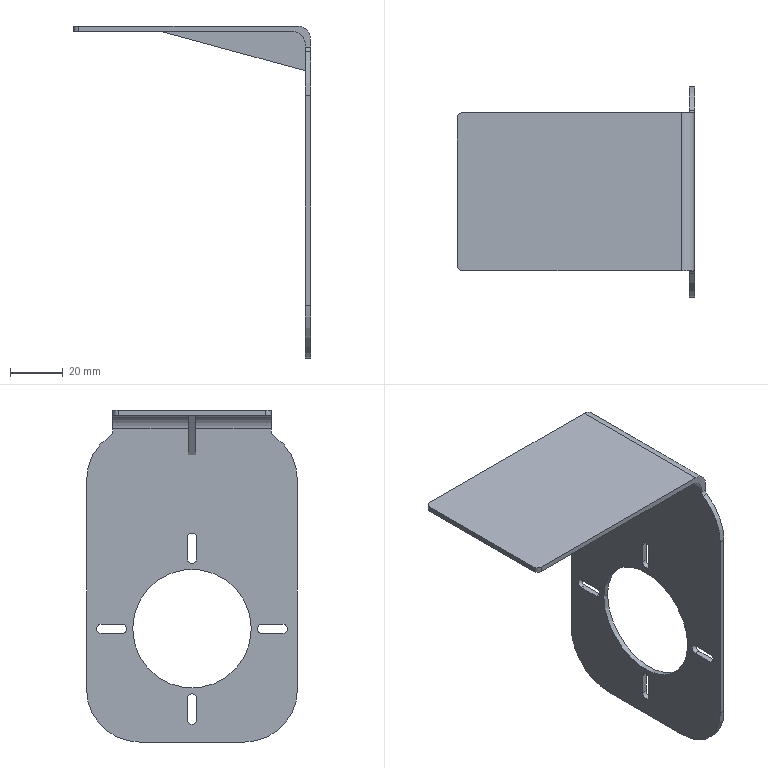Component | SolidWorks | ImagingSystem-1111-1_123456789-DL-OP20-ST12--004-1111-1 | 1 solid | 43 faces | box 90 x 80 x 126 mm | volume 27547 mm3 | cylinder 22 | plane 21 | commonest cylinder face diameters 3.5 x9 4 x4 40 x4 10 x3 45 x2 | material AL6061
build123d program:
from build123d import *

# Parameters (mm, degrees)
SKETCH1_W                  = 80
SKETCH1_H                  = 126
BOSS_EXTRUDE1_DEPTH        = 30
SKETCH2_W                  = 20
SKETCH2_H                  = 116
CUT_EXTRUDE1_DEPTH         = 152.331
F_25_0_25_DIAMETER_HOLE1_D = 45
CHAMFER1_SIZE              = 2
SKETCH9_W                  = 30
SKETCH9_H                  = 10
CUT_EXTRUDE3_DEPTH         = 10
SKETCH10_W                 = 30
SKETCH10_H                 = 10
CUT_EXTRUDE4_DEPTH         = 10
MOVE_FACE1_BY              = 3
MOVE_FACE1_2_BY            = 3
SKETCH15_W                 = 3
SKETCH15_H                 = 30
BOSS_EXTRUDE2_DEPTH        = 3
F_3_5_3_5_DIAMETER_HOLE2_D = 3.5
CIRPATTERN1_COUNT          = 4
MOVE_FACE2_BY              = 8
SKETCH22_W                 = 30
SKETCH22_H                 = 3
CUT_EXTRUDE11_DEPTH        = 10
SKETCH23_W                 = 30
SKETCH23_H                 = 3
CUT_EXTRUDE12_DEPTH        = 10
MOVE_FACE4_BY              = 8
FILLET3_R                  = 5
MOVE_FACE6_BY              = 3
MOVE_FACE7_BY              = 3
MOVE_FACE8_BY              = 60
FILLET4_R                  = 2
FILLET8_R                  = 20
BOSS_EXTRUDE7_DEPTH        = 1.5
CUT_EXTRUDE15_DEPTH        = 174.263
CIRPATTERN2_COUNT          = 4


with BuildPart() as part:
    # Sketch1 → Boss-Extrude1 (new body)
    with BuildSketch(Plane.XY.offset(25)):
        with Locations((40, 63)):
            Rectangle(SKETCH1_W, SKETCH1_H)
    extrude(amount=-BOSS_EXTRUDE1_DEPTH)

    # Sketch2 → Cut-Extrude1 (cut, through all)
    with BuildSketch(Plane.ZY):
        with Locations((15, 58)):
            Rectangle(SKETCH2_W, SKETCH2_H)
    extrude(amount=-CUT_EXTRUDE1_DEPTH, mode=Mode.SUBTRACT)

    # 25.0 _25_ Diameter Hole1 (through all)
    with Locations(Plane.XY.offset(5)):
        with Locations((40, 43)):
            Hole(F_25_0_25_DIAMETER_HOLE1_D / 2)

    # Chamfer1
    chamfer1_edges = [part.edges().sort_by_distance(p)[0] for p in [
        (80, 121, 25),
        (0, 121, 25),
    ]]
    chamfer(chamfer1_edges, length=CHAMFER1_SIZE)

    # Sketch9 → Cut-Extrude3 (cut)
    with BuildSketch(Plane(origin=(80, 0, 0), x_dir=(0, 0, -1), z_dir=(1, 0, 0))):
        with Locations((-10, 121)):
            Rectangle(SKETCH9_W, SKETCH9_H)
    extrude(amount=-CUT_EXTRUDE3_DEPTH, mode=Mode.SUBTRACT)

    # Sketch10 → Cut-Extrude4 (cut)
    with BuildSketch(Plane.ZY):
        with Locations((10, 121)):
            Rectangle(SKETCH10_W, SKETCH10_H)
    extrude(amount=-CUT_EXTRUDE4_DEPTH, mode=Mode.SUBTRACT)

    # Move Face1: a face moved outward by 3.0
    extrude(part.faces().sort_by_distance((10, 121, 10))[0], amount=MOVE_FACE1_BY, dir=(-1, 0, 0))

    # Move Face1 2: a face moved outward by 3.0
    extrude(part.faces().sort_by_distance((70, 121, 10))[0], amount=MOVE_FACE1_2_BY, dir=(1, 0, 0))

    # Sketch15 → Boss-Extrude2 (add)
    with BuildSketch(Plane(origin=(0, 126, 0), x_dir=(1, 0, 0), z_dir=(0, 1, 0))):
        with Locations((8.5, -10)):
            Rectangle(SKETCH15_W, SKETCH15_H)
        with Locations((71.5, -10)):
            Rectangle(SKETCH15_W, SKETCH15_H)
    extrude(amount=BOSS_EXTRUDE2_DEPTH)

    # Sketch18 → 3.5 _3.5_ Diameter Hole1 (revolve, cut)
    with BuildSketch(Plane(origin=(40, 77.5, 5), x_dir=(0, -1, 0), z_dir=(1, 0, 0))):
        Polygon((0, 0), (0, 31.052), (1.75, 30), (1.75, 0), align=None)
    f_3_5_3_5_diameter_hole1 = revolve(axis=Axis((40, 77.5, 11.35), (0, 0, -1)), mode=Mode.SUBTRACT)

    # 3.5 _3.5_ Diameter Hole2 (through all)
    with Locations(Plane.XY.offset(5)):
        with Locations((40, 73)):
            f_3_5_3_5_diameter_hole2 = Hole(F_3_5_3_5_DIAMETER_HOLE2_D / 2)

    # CirPattern1: 3.5 _3.5_ Diameter Hole1, 3.5 _3.5_ Diameter Hole2 ×4 about axis
    cirpattern1_axis = Axis((40, 43, 0), (0, 0, 1))
    add([f_3_5_3_5_diameter_hole1.rotate(cirpattern1_axis, i * 360 / CIRPATTERN1_COUNT) for i in range(1, CIRPATTERN1_COUNT)], mode=Mode.SUBTRACT)
    add([f_3_5_3_5_diameter_hole2.rotate(cirpattern1_axis, i * 360 / CIRPATTERN1_COUNT) for i in range(1, CIRPATTERN1_COUNT)], mode=Mode.SUBTRACT)

    # Move Face2: a face moved inward by 8.0
    extrude(part.faces().sort_by_distance((40, 116, 15))[0], amount=MOVE_FACE2_BY, dir=(0, 1, 0), mode=Mode.SUBTRACT)

    # Sketch22 → Cut-Extrude11 (cut)
    with BuildSketch(Plane(origin=(10, 0, 0), x_dir=(0, 0, -1), z_dir=(1, 0, 0))):
        with Locations((-10, 127.5)):
            Rectangle(SKETCH22_W, SKETCH22_H)
    extrude(amount=-CUT_EXTRUDE11_DEPTH, mode=Mode.SUBTRACT)

    # Sketch23 → Cut-Extrude12 (cut)
    with BuildSketch(Plane.ZY.offset(-70)):
        with Locations((10, 127.5)):
            Rectangle(SKETCH23_W, SKETCH23_H)
    extrude(amount=-CUT_EXTRUDE12_DEPTH, mode=Mode.SUBTRACT)

    # Move Face4: a face moved inward by 8.0
    extrude(part.faces().sort_by_distance((60, 62, 5))[0], amount=MOVE_FACE4_BY, dir=(0, 0, -1), mode=Mode.SUBTRACT)

    # Fillet3
    fillet3_edges = [part.edges().sort_by_distance(p)[0] for p in [
        (40, 126, -5),
        (40, 124, -3),
    ]]
    fillet(fillet3_edges, radius=FILLET3_R)

    # Move Face6: a face moved inward by 3.0
    extrude(part.faces().sort_by_distance((7, 125, 10))[0], amount=MOVE_FACE6_BY, dir=(1, 0, 0), mode=Mode.SUBTRACT)

    # Move Face7: a face moved inward by 3.0
    extrude(part.faces().sort_by_distance((73, 125, 10))[0], amount=MOVE_FACE7_BY, dir=(-1, 0, 0), mode=Mode.SUBTRACT)

    # Move Face8: a face moved outward by 60.0
    extrude(part.faces().sort_by_distance((40, 125, 25))[0], amount=MOVE_FACE8_BY, dir=(0, 0, 1))

    # Fillet4
    fillet4_edges = [part.edges().sort_by_distance(p)[0] for p in [
        (70, 125, 85),
        (70, 116, -4),
        (10, 116, -4),
        (10, 125, 85),
    ]]
    fillet(fillet4_edges, radius=FILLET4_R)

    # Fillet8
    fillet8_edges = [part.edges().sort_by_distance(p)[0] for p in [
        (0, 116, -4),
        (80, 116, -4),
        (80, 0, -4),
        (0, 0, -4),
    ]]
    fillet(fillet8_edges, radius=FILLET8_R)

    # Sketch35 → Boss-Extrude7 (add, symmetric)
    with BuildSketch(Plane(origin=(40, 0, 0), x_dir=(0, 0, -1), z_dir=(1, 0, 0))):
        with BuildLine():
            Line((3, 116.324), (3, 109))
            Line((3, 109), (-52, 124))
            Line((-52, 124), (-2, 124))
            ThreePointArc((-2, 124), (1.536, 122.536), (3, 119))
            Line((3, 119), (3, 118))
            Line((3, 118), (3, 116.324))
        make_face()
    extrude(amount=BOSS_EXTRUDE7_DEPTH, both=True)

    # Sketch36 → Cut-Extrude15 (cut, through all)
    with BuildSketch(Plane.XY.offset(-3)):
        with BuildLine():
            Line((41.75, 77.5), (41.75, 69.5))
            ThreePointArc((41.75, 69.5), (40, 67.75), (38.25, 69.5))
            Line((38.25, 69.5), (38.25, 77.5))
            ThreePointArc((38.25, 77.5), (40, 79.25), (41.75, 77.5))
        make_face()
    cut_extrude15 = extrude(amount=-CUT_EXTRUDE15_DEPTH, mode=Mode.SUBTRACT)

    # CirPattern2: Cut-Extrude15 ×4 about axis
    cirpattern2_axis = Axis((40, 43, 0), (0, 0, 1))
    for i in range(1, CIRPATTERN2_COUNT):
        add(cut_extrude15.rotate(cirpattern2_axis, i * 360 / CIRPATTERN2_COUNT), mode=Mode.SUBTRACT)


solid = part.part

# Placed as in the assembly
solid = solid.moved(Location((169.441, -15, -118), (90, -90, 0)))